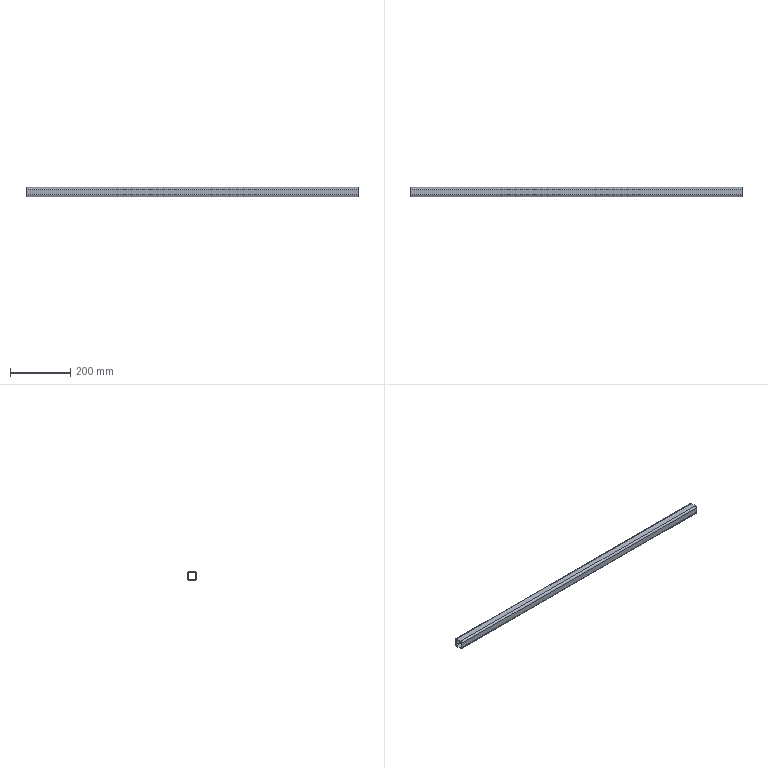Component | SolidWorks | 30X30X3-1100-3 | 1 solid | 18 faces | box 1100 x 30 x 30 mm | volume 330905 mm3 | plane 10 | cylinder 8 | commonest cylinder face diameters 12 x4 6 x4
build123d program:
from build123d import *

# Parameters (mm, degrees)
GB_6728_1986_SQUARE_HOLLOW_SECTION_030_X_DEPTH = 1100


with BuildPart() as part:
    # Sketch1 → Gb_6728-1986 Square Hollow Section 030 X (new body)
    with BuildSketch(Plane(origin=(0, 0, 0), x_dir=(-1, 0, 0), z_dir=(0, 1, 0))):
        with BuildLine():
            Line((-9, -15), (9, -15))
            ThreePointArc((9, -15), (13.243, -13.243), (15, -9))
            Line((15, -9), (15, 9))
            ThreePointArc((15, 9), (13.243, 13.243), (9, 15))
            Line((9, 15), (-9, 15))
            ThreePointArc((-9, 15), (-13.243, 13.243), (-15, 9))
            Line((-15, 9), (-15, -9))
            ThreePointArc((-15, -9), (-13.243, -13.243), (-9, -15))
        make_face()
        with BuildLine():
            Line((-9, -12), (9, -12))
            ThreePointArc((9, -12), (11.121, -11.121), (12, -9))
            Line((12, -9), (12, 9))
            ThreePointArc((12, 9), (11.121, 11.121), (9, 12))
            Line((9, 12), (-9, 12))
            ThreePointArc((-9, 12), (-11.121, 11.121), (-12, 9))
            Line((-12, 9), (-12, -9))
            ThreePointArc((-12, -9), (-11.121, -11.121), (-9, -12))
        make_face(mode=Mode.SUBTRACT)
    extrude(amount=GB_6728_1986_SQUARE_HOLLOW_SECTION_030_X_DEPTH)


solid = part.part

# Placed as in the assembly
solid = solid.moved(Location((3169.926, -31179.846, 5264), (0, 0, 90)))
STEP:
#1=COLOUR_RGB('',0.7922,0.8196,0.9333);
#2=FILL_AREA_STYLE_COLOUR('',#1);
#3=FILL_AREA_STYLE('',(#2));
#4=SURFACE_STYLE_FILL_AREA(#3);
#5=SURFACE_SIDE_STYLE('',(#4));
#6=SURFACE_STYLE_USAGE(.BOTH.,#5);
#7=PRESENTATION_STYLE_ASSIGNMENT((#6));
#8=CARTESIAN_POINT('',(81.493,-1227.199,206.654));
#9=VERTEX_POINT('',#8);
#10=CARTESIAN_POINT('',(81.493,-1226.962,206.89));
#11=VERTEX_POINT('',#10);
#12=CARTESIAN_POINT('',(81.493,-1227.199,206.89));
#13=DIRECTION('',(1.,-0.,-0.));
#14=DIRECTION('',(0.,1.,0.));
#15=AXIS2_PLACEMENT_3D('',#12,#13,#14);
#16=CIRCLE('',#15,0.2362);
#17=EDGE_CURVE('',#9,#11,#16,.T.);
#18=ORIENTED_EDGE('',*,*,#17,.T.);
#19=CARTESIAN_POINT('',(124.8,-1226.962,206.89));
#20=VERTEX_POINT('',#19);
#21=CARTESIAN_POINT('',(124.8,-1226.962,206.89));
#22=DIRECTION('',(-1.,0.,0.));
#23=VECTOR('',#22,39.37);
#24=LINE('',#21,#23);
#25=EDGE_CURVE('',#20,#11,#24,.T.);
#26=ORIENTED_EDGE('',*,*,#25,.F.);
#27=CARTESIAN_POINT('',(124.8,-1227.199,206.654));
#28=VERTEX_POINT('',#27);
#29=CARTESIAN_POINT('',(124.8,-1227.199,206.89));
#30=DIRECTION('',(1.,-0.,-0.));
#31=DIRECTION('',(0.,1.,0.));
#32=AXIS2_PLACEMENT_3D('',#29,#30,#31);
#33=CIRCLE('',#32,0.2362);
#34=EDGE_CURVE('',#28,#20,#33,.T.);
#35=ORIENTED_EDGE('',*,*,#34,.F.);
#36=CARTESIAN_POINT('',(124.8,-1227.199,206.654));
#37=DIRECTION('',(-1.,0.,0.));
#38=VECTOR('',#37,39.37);
#39=LINE('',#36,#38);
#40=EDGE_CURVE('',#28,#9,#39,.T.);
#41=ORIENTED_EDGE('',*,*,#40,.T.);
#42=EDGE_LOOP('',(#18,#26,#35,#41));
#43=FACE_OUTER_BOUND('',#42,.T.);
#44=CARTESIAN_POINT('',(124.8,-1227.199,206.89));
#45=DIRECTION('',(-1.,0.,0.));
#46=DIRECTION('',(0.,-1.,0.));
#47=AXIS2_PLACEMENT_3D('',#44,#45,#46);
#48=CYLINDRICAL_SURFACE('',#47,0.2362);
#49=ADVANCED_FACE('',(#43),#48,.T.);
#50=CARTESIAN_POINT('',(81.493,-1226.962,207.598));
#51=VERTEX_POINT('',#50);
#52=CARTESIAN_POINT('',(81.493,-1226.962,206.89));
#53=DIRECTION('',(0.,-0.,1.));
#54=VECTOR('',#53,39.37);
#55=LINE('',#52,#54);
#56=EDGE_CURVE('',#11,#51,#55,.T.);
#57=ORIENTED_EDGE('',*,*,#56,.T.);
#58=CARTESIAN_POINT('',(124.8,-1226.962,207.598));
#59=VERTEX_POINT('',#58);
#60=CARTESIAN_POINT('',(124.8,-1226.962,207.598));
#61=DIRECTION('',(-1.,0.,0.));
#62=VECTOR('',#61,39.37);
#63=LINE('',#60,#62);
#64=EDGE_CURVE('',#59,#51,#63,.T.);
#65=ORIENTED_EDGE('',*,*,#64,.F.);
#66=CARTESIAN_POINT('',(124.8,-1226.962,206.89));
#67=DIRECTION('',(0.,-0.,1.));
#68=VECTOR('',#67,39.37);
#69=LINE('',#66,#68);
#70=EDGE_CURVE('',#20,#59,#69,.T.);
#71=ORIENTED_EDGE('',*,*,#70,.F.);
#72=ORIENTED_EDGE('',*,*,#25,.T.);
#73=EDGE_LOOP('',(#57,#65,#71,#72));
#74=FACE_OUTER_BOUND('',#73,.T.);
#75=CARTESIAN_POINT('',(124.8,-1226.962,206.89));
#76=DIRECTION('',(-0.,-1.,-0.));
#77=DIRECTION('',(-0.,0.,-1.));
#78=AXIS2_PLACEMENT_3D('',#75,#76,#77);
#79=PLANE('',#78);
#80=ADVANCED_FACE('',(#74),#79,.F.);
#81=CARTESIAN_POINT('',(81.493,-1227.199,207.835));
#82=VERTEX_POINT('',#81);
#83=CARTESIAN_POINT('',(81.493,-1227.199,207.598));
#84=DIRECTION('',(1.,-0.,-0.));
#85=DIRECTION('',(0.,1.,0.));
#86=AXIS2_PLACEMENT_3D('',#83,#84,#85);
#87=CIRCLE('',#86,0.2362);
#88=EDGE_CURVE('',#51,#82,#87,.T.);
#89=ORIENTED_EDGE('',*,*,#88,.T.);
#90=CARTESIAN_POINT('',(124.8,-1227.199,207.835));
#91=VERTEX_POINT('',#90);
#92=CARTESIAN_POINT('',(124.8,-1227.199,207.835));
#93=DIRECTION('',(-1.,0.,0.));
#94=VECTOR('',#93,39.37);
#95=LINE('',#92,#94);
#96=EDGE_CURVE('',#91,#82,#95,.T.);
#97=ORIENTED_EDGE('',*,*,#96,.F.);
#98=CARTESIAN_POINT('',(124.8,-1227.199,207.598));
#99=DIRECTION('',(1.,-0.,-0.));
#100=DIRECTION('',(0.,1.,0.));
#101=AXIS2_PLACEMENT_3D('',#98,#99,#100);
#102=CIRCLE('',#101,0.2362);
#103=EDGE_CURVE('',#59,#91,#102,.T.);
#104=ORIENTED_EDGE('',*,*,#103,.F.);
#105=ORIENTED_EDGE('',*,*,#64,.T.);
#106=EDGE_LOOP('',(#89,#97,#104,#105));
#107=FACE_OUTER_BOUND('',#106,.T.);
#108=CARTESIAN_POINT('',(124.8,-1227.199,207.598));
#109=DIRECTION('',(-1.,0.,0.));
#110=DIRECTION('',(0.,-1.,0.));
#111=AXIS2_PLACEMENT_3D('',#108,#109,#110);
#112=CYLINDRICAL_SURFACE('',#111,0.2362);
#113=ADVANCED_FACE('',(#107),#112,.T.);
#114=CARTESIAN_POINT('',(81.493,-1227.907,207.835));
#115=VERTEX_POINT('',#114);
#116=CARTESIAN_POINT('',(81.493,-1227.907,207.835));
#117=DIRECTION('',(-0.,-1.,-0.));
#118=VECTOR('',#117,39.37);
#119=LINE('',#116,#118);
#120=EDGE_CURVE('',#82,#115,#119,.T.);
#121=ORIENTED_EDGE('',*,*,#120,.T.);
#122=CARTESIAN_POINT('',(124.8,-1227.907,207.835));
#123=VERTEX_POINT('',#122);
#124=CARTESIAN_POINT('',(124.8,-1227.907,207.835));
#125=DIRECTION('',(-1.,0.,0.));
#126=VECTOR('',#125,39.37);
#127=LINE('',#124,#126);
#128=EDGE_CURVE('',#123,#115,#127,.T.);
#129=ORIENTED_EDGE('',*,*,#128,.F.);
#130=CARTESIAN_POINT('',(124.8,-1227.907,207.835));
#131=DIRECTION('',(-0.,-1.,-0.));
#132=VECTOR('',#131,39.37);
#133=LINE('',#130,#132);
#134=EDGE_CURVE('',#91,#123,#133,.T.);
#135=ORIENTED_EDGE('',*,*,#134,.F.);
#136=ORIENTED_EDGE('',*,*,#96,.T.);
#137=EDGE_LOOP('',(#121,#129,#135,#136));
#138=FACE_OUTER_BOUND('',#137,.T.);
#139=CARTESIAN_POINT('',(124.8,-1227.907,207.835));
#140=DIRECTION('',(-0.,0.,-1.));
#141=DIRECTION('',(0.,1.,0.));
#142=AXIS2_PLACEMENT_3D('',#139,#140,#141);
#143=PLANE('',#142);
#144=ADVANCED_FACE('',(#138),#143,.F.);
#145=CARTESIAN_POINT('',(81.493,-1228.144,207.598));
#146=VERTEX_POINT('',#145);
#147=CARTESIAN_POINT('',(81.493,-1227.907,207.598));
#148=DIRECTION('',(1.,-0.,-0.));
#149=DIRECTION('',(0.,1.,0.));
#150=AXIS2_PLACEMENT_3D('',#147,#148,#149);
#151=CIRCLE('',#150,0.2362);
#152=EDGE_CURVE('',#115,#146,#151,.T.);
#153=ORIENTED_EDGE('',*,*,#152,.T.);
#154=CARTESIAN_POINT('',(124.8,-1228.144,207.598));
#155=VERTEX_POINT('',#154);
#156=CARTESIAN_POINT('',(124.8,-1228.144,207.598));
#157=DIRECTION('',(-1.,0.,0.));
#158=VECTOR('',#157,39.37);
#159=LINE('',#156,#158);
#160=EDGE_CURVE('',#155,#146,#159,.T.);
#161=ORIENTED_EDGE('',*,*,#160,.F.);
#162=CARTESIAN_POINT('',(124.8,-1227.907,207.598));
#163=DIRECTION('',(1.,-0.,-0.));
#164=DIRECTION('',(0.,1.,0.));
#165=AXIS2_PLACEMENT_3D('',#162,#163,#164);
#166=CIRCLE('',#165,0.2362);
#167=EDGE_CURVE('',#123,#155,#166,.T.);
#168=ORIENTED_EDGE('',*,*,#167,.F.);
#169=ORIENTED_EDGE('',*,*,#128,.T.);
#170=EDGE_LOOP('',(#153,#161,#168,#169));
#171=FACE_OUTER_BOUND('',#170,.T.);
#172=CARTESIAN_POINT('',(124.8,-1227.907,207.598));
#173=DIRECTION('',(-1.,0.,0.));
#174=DIRECTION('',(0.,-1.,0.));
#175=AXIS2_PLACEMENT_3D('',#172,#173,#174);
#176=CYLINDRICAL_SURFACE('',#175,0.2362);
#177=ADVANCED_FACE('',(#171),#176,.T.);
#178=CARTESIAN_POINT('',(81.493,-1228.144,206.89));
#179=VERTEX_POINT('',#178);
#180=CARTESIAN_POINT('',(81.493,-1228.144,207.598));
#181=DIRECTION('',(-0.,0.,-1.));
#182=VECTOR('',#181,39.37);
#183=LINE('',#180,#182);
#184=EDGE_CURVE('',#146,#179,#183,.T.);
#185=ORIENTED_EDGE('',*,*,#184,.T.);
#186=CARTESIAN_POINT('',(124.8,-1228.144,206.89));
#187=VERTEX_POINT('',#186);
#188=CARTESIAN_POINT('',(124.8,-1228.144,206.89));
#189=DIRECTION('',(-1.,0.,0.));
#190=VECTOR('',#189,39.37);
#191=LINE('',#188,#190);
#192=EDGE_CURVE('',#187,#179,#191,.T.);
#193=ORIENTED_EDGE('',*,*,#192,.F.);
#194=CARTESIAN_POINT('',(124.8,-1228.144,207.598));
#195=DIRECTION('',(-0.,0.,-1.));
#196=VECTOR('',#195,39.37);
#197=LINE('',#194,#196);
#198=EDGE_CURVE('',#155,#187,#197,.T.);
#199=ORIENTED_EDGE('',*,*,#198,.F.);
#200=ORIENTED_EDGE('',*,*,#160,.T.);
#201=EDGE_LOOP('',(#185,#193,#199,#200));
#202=FACE_OUTER_BOUND('',#201,.T.);
#203=CARTESIAN_POINT('',(124.8,-1228.144,207.598));
#204=DIRECTION('',(0.,1.,0.));
#205=DIRECTION('',(0.,-0.,1.));
#206=AXIS2_PLACEMENT_3D('',#203,#204,#205);
#207=PLANE('',#206);
#208=ADVANCED_FACE('',(#202),#207,.F.);
#209=CARTESIAN_POINT('',(81.493,-1227.907,206.654));
#210=VERTEX_POINT('',#209);
#211=CARTESIAN_POINT('',(81.493,-1227.907,206.89));
#212=DIRECTION('',(1.,-0.,-0.));
#213=DIRECTION('',(0.,1.,0.));
#214=AXIS2_PLACEMENT_3D('',#211,#212,#213);
#215=CIRCLE('',#214,0.2362);
#216=EDGE_CURVE('',#179,#210,#215,.T.);
#217=ORIENTED_EDGE('',*,*,#216,.T.);
#218=CARTESIAN_POINT('',(124.8,-1227.907,206.654));
#219=VERTEX_POINT('',#218);
#220=CARTESIAN_POINT('',(124.8,-1227.907,206.654));
#221=DIRECTION('',(-1.,0.,0.));
#222=VECTOR('',#221,39.37);
#223=LINE('',#220,#222);
#224=EDGE_CURVE('',#219,#210,#223,.T.);
#225=ORIENTED_EDGE('',*,*,#224,.F.);
#226=CARTESIAN_POINT('',(124.8,-1227.907,206.89));
#227=DIRECTION('',(1.,-0.,-0.));
#228=DIRECTION('',(0.,1.,0.));
#229=AXIS2_PLACEMENT_3D('',#226,#227,#228);
#230=CIRCLE('',#229,0.2362);
#231=EDGE_CURVE('',#187,#219,#230,.T.);
#232=ORIENTED_EDGE('',*,*,#231,.F.);
#233=ORIENTED_EDGE('',*,*,#192,.T.);
#234=EDGE_LOOP('',(#217,#225,#232,#233));
#235=FACE_OUTER_BOUND('',#234,.T.);
#236=CARTESIAN_POINT('',(124.8,-1227.907,206.89));
#237=DIRECTION('',(-1.,0.,0.));
#238=DIRECTION('',(0.,-1.,0.));
#239=AXIS2_PLACEMENT_3D('',#236,#237,#238);
#240=CYLINDRICAL_SURFACE('',#239,0.2362);
#241=ADVANCED_FACE('',(#235),#240,.T.);
#242=CARTESIAN_POINT('',(81.493,-1227.081,207.598));
#243=VERTEX_POINT('',#242);
#244=CARTESIAN_POINT('',(81.493,-1227.199,207.717));
#245=VERTEX_POINT('',#244);
#246=CARTESIAN_POINT('',(81.493,-1227.199,207.598));
#247=DIRECTION('',(1.,-0.,-0.));
#248=DIRECTION('',(0.,1.,0.));
#249=AXIS2_PLACEMENT_3D('',#246,#247,#248);
#250=CIRCLE('',#249,0.1181);
#251=EDGE_CURVE('',#243,#245,#250,.T.);
#252=ORIENTED_EDGE('',*,*,#251,.F.);
#253=CARTESIAN_POINT('',(124.8,-1227.081,207.598));
#254=VERTEX_POINT('',#253);
#255=CARTESIAN_POINT('',(124.8,-1227.081,207.598));
#256=DIRECTION('',(-1.,0.,0.));
#257=VECTOR('',#256,39.37);
#258=LINE('',#255,#257);
#259=EDGE_CURVE('',#254,#243,#258,.T.);
#260=ORIENTED_EDGE('',*,*,#259,.F.);
#261=CARTESIAN_POINT('',(124.8,-1227.199,207.717));
#262=VERTEX_POINT('',#261);
#263=CARTESIAN_POINT('',(124.8,-1227.199,207.598));
#264=DIRECTION('',(1.,-0.,-0.));
#265=DIRECTION('',(0.,1.,0.));
#266=AXIS2_PLACEMENT_3D('',#263,#264,#265);
#267=CIRCLE('',#266,0.1181);
#268=EDGE_CURVE('',#254,#262,#267,.T.);
#269=ORIENTED_EDGE('',*,*,#268,.T.);
#270=CARTESIAN_POINT('',(124.8,-1227.199,207.717));
#271=DIRECTION('',(-1.,0.,0.));
#272=VECTOR('',#271,39.37);
#273=LINE('',#270,#272);
#274=EDGE_CURVE('',#262,#245,#273,.T.);
#275=ORIENTED_EDGE('',*,*,#274,.T.);
#276=EDGE_LOOP('',(#252,#260,#269,#275));
#277=FACE_OUTER_BOUND('',#276,.T.);
#278=CARTESIAN_POINT('',(124.8,-1227.199,207.598));
#279=DIRECTION('',(-1.,0.,0.));
#280=DIRECTION('',(0.,-1.,0.));
#281=AXIS2_PLACEMENT_3D('',#278,#279,#280);
#282=CYLINDRICAL_SURFACE('',#281,0.1181);
#283=ADVANCED_FACE('',(#277),#282,.F.);
#284=CARTESIAN_POINT('',(81.493,-1227.081,206.89));
#285=VERTEX_POINT('',#284);
#286=CARTESIAN_POINT('',(81.493,-1227.081,206.89));
#287=DIRECTION('',(0.,-0.,1.));
#288=VECTOR('',#287,39.37);
#289=LINE('',#286,#288);
#290=EDGE_CURVE('',#285,#243,#289,.T.);
#291=ORIENTED_EDGE('',*,*,#290,.F.);
#292=CARTESIAN_POINT('',(124.8,-1227.081,206.89));
#293=VERTEX_POINT('',#292);
#294=CARTESIAN_POINT('',(124.8,-1227.081,206.89));
#295=DIRECTION('',(-1.,0.,0.));
#296=VECTOR('',#295,39.37);
#297=LINE('',#294,#296);
#298=EDGE_CURVE('',#293,#285,#297,.T.);
#299=ORIENTED_EDGE('',*,*,#298,.F.);
#300=CARTESIAN_POINT('',(124.8,-1227.081,206.89));
#301=DIRECTION('',(0.,-0.,1.));
#302=VECTOR('',#301,39.37);
#303=LINE('',#300,#302);
#304=EDGE_CURVE('',#293,#254,#303,.T.);
#305=ORIENTED_EDGE('',*,*,#304,.T.);
#306=ORIENTED_EDGE('',*,*,#259,.T.);
#307=EDGE_LOOP('',(#291,#299,#305,#306));
#308=FACE_OUTER_BOUND('',#307,.T.);
#309=CARTESIAN_POINT('',(124.8,-1227.081,206.89));
#310=DIRECTION('',(-0.,-1.,-0.));
#311=DIRECTION('',(-0.,0.,-1.));
#312=AXIS2_PLACEMENT_3D('',#309,#310,#311);
#313=PLANE('',#312);
#314=ADVANCED_FACE('',(#308),#313,.T.);
#315=CARTESIAN_POINT('',(81.493,-1227.199,206.772));
#316=VERTEX_POINT('',#315);
#317=CARTESIAN_POINT('',(81.493,-1227.199,206.89));
#318=DIRECTION('',(1.,-0.,-0.));
#319=DIRECTION('',(0.,1.,0.));
#320=AXIS2_PLACEMENT_3D('',#317,#318,#319);
#321=CIRCLE('',#320,0.1181);
#322=EDGE_CURVE('',#316,#285,#321,.T.);
#323=ORIENTED_EDGE('',*,*,#322,.F.);
#324=CARTESIAN_POINT('',(124.8,-1227.199,206.772));
#325=VERTEX_POINT('',#324);
#326=CARTESIAN_POINT('',(124.8,-1227.199,206.772));
#327=DIRECTION('',(-1.,0.,0.));
#328=VECTOR('',#327,39.37);
#329=LINE('',#326,#328);
#330=EDGE_CURVE('',#325,#316,#329,.T.);
#331=ORIENTED_EDGE('',*,*,#330,.F.);
#332=CARTESIAN_POINT('',(124.8,-1227.199,206.89));
#333=DIRECTION('',(1.,-0.,-0.));
#334=DIRECTION('',(0.,1.,0.));
#335=AXIS2_PLACEMENT_3D('',#332,#333,#334);
#336=CIRCLE('',#335,0.1181);
#337=EDGE_CURVE('',#325,#293,#336,.T.);
#338=ORIENTED_EDGE('',*,*,#337,.T.);
#339=ORIENTED_EDGE('',*,*,#298,.T.);
#340=EDGE_LOOP('',(#323,#331,#338,#339));
#341=FACE_OUTER_BOUND('',#340,.T.);
#342=CARTESIAN_POINT('',(124.8,-1227.199,206.89));
#343=DIRECTION('',(-1.,0.,0.));
#344=DIRECTION('',(0.,-1.,0.));
#345=AXIS2_PLACEMENT_3D('',#342,#343,#344);
#346=CYLINDRICAL_SURFACE('',#345,0.1181);
#347=ADVANCED_FACE('',(#341),#346,.F.);
#348=CARTESIAN_POINT('',(81.493,-1227.907,206.772));
#349=VERTEX_POINT('',#348);
#350=CARTESIAN_POINT('',(81.493,-1227.199,206.772));
#351=DIRECTION('',(0.,1.,0.));
#352=VECTOR('',#351,39.37);
#353=LINE('',#350,#352);
#354=EDGE_CURVE('',#349,#316,#353,.T.);
#355=ORIENTED_EDGE('',*,*,#354,.F.);
#356=CARTESIAN_POINT('',(124.8,-1227.907,206.772));
#357=VERTEX_POINT('',#356);
#358=CARTESIAN_POINT('',(124.8,-1227.907,206.772));
#359=DIRECTION('',(-1.,0.,0.));
#360=VECTOR('',#359,39.37);
#361=LINE('',#358,#360);
#362=EDGE_CURVE('',#357,#349,#361,.T.);
#363=ORIENTED_EDGE('',*,*,#362,.F.);
#364=CARTESIAN_POINT('',(124.8,-1227.199,206.772));
#365=DIRECTION('',(0.,1.,0.));
#366=VECTOR('',#365,39.37);
#367=LINE('',#364,#366);
#368=EDGE_CURVE('',#357,#325,#367,.T.);
#369=ORIENTED_EDGE('',*,*,#368,.T.);
#370=ORIENTED_EDGE('',*,*,#330,.T.);
#371=EDGE_LOOP('',(#355,#363,#369,#370));
#372=FACE_OUTER_BOUND('',#371,.T.);
#373=CARTESIAN_POINT('',(124.8,-1227.199,206.772));
#374=DIRECTION('',(0.,-0.,1.));
#375=DIRECTION('',(-0.,-1.,-0.));
#376=AXIS2_PLACEMENT_3D('',#373,#374,#375);
#377=PLANE('',#376);
#378=ADVANCED_FACE('',(#372),#377,.T.);
#379=CARTESIAN_POINT('',(81.493,-1228.025,206.89));
#380=VERTEX_POINT('',#379);
#381=CARTESIAN_POINT('',(81.493,-1227.907,206.89));
#382=DIRECTION('',(1.,-0.,-0.));
#383=DIRECTION('',(0.,1.,0.));
#384=AXIS2_PLACEMENT_3D('',#381,#382,#383);
#385=CIRCLE('',#384,0.1181);
#386=EDGE_CURVE('',#380,#349,#385,.T.);
#387=ORIENTED_EDGE('',*,*,#386,.F.);
#388=CARTESIAN_POINT('',(124.8,-1228.025,206.89));
#389=VERTEX_POINT('',#388);
#390=CARTESIAN_POINT('',(124.8,-1228.025,206.89));
#391=DIRECTION('',(-1.,0.,0.));
#392=VECTOR('',#391,39.37);
#393=LINE('',#390,#392);
#394=EDGE_CURVE('',#389,#380,#393,.T.);
#395=ORIENTED_EDGE('',*,*,#394,.F.);
#396=CARTESIAN_POINT('',(124.8,-1227.907,206.89));
#397=DIRECTION('',(1.,-0.,-0.));
#398=DIRECTION('',(0.,1.,0.));
#399=AXIS2_PLACEMENT_3D('',#396,#397,#398);
#400=CIRCLE('',#399,0.1181);
#401=EDGE_CURVE('',#389,#357,#400,.T.);
#402=ORIENTED_EDGE('',*,*,#401,.T.);
#403=ORIENTED_EDGE('',*,*,#362,.T.);
#404=EDGE_LOOP('',(#387,#395,#402,#403));
#405=FACE_OUTER_BOUND('',#404,.T.);
#406=CARTESIAN_POINT('',(124.8,-1227.907,206.89));
#407=DIRECTION('',(-1.,0.,0.));
#408=DIRECTION('',(0.,-1.,0.));
#409=AXIS2_PLACEMENT_3D('',#406,#407,#408);
#410=CYLINDRICAL_SURFACE('',#409,0.1181);
#411=ADVANCED_FACE('',(#405),#410,.F.);
#412=CARTESIAN_POINT('',(81.493,-1228.025,207.598));
#413=VERTEX_POINT('',#412);
#414=CARTESIAN_POINT('',(81.493,-1228.025,207.598));
#415=DIRECTION('',(-0.,0.,-1.));
#416=VECTOR('',#415,39.37);
#417=LINE('',#414,#416);
#418=EDGE_CURVE('',#413,#380,#417,.T.);
#419=ORIENTED_EDGE('',*,*,#418,.F.);
#420=CARTESIAN_POINT('',(124.8,-1228.025,207.598));
#421=VERTEX_POINT('',#420);
#422=CARTESIAN_POINT('',(124.8,-1228.025,207.598));
#423=DIRECTION('',(-1.,0.,0.));
#424=VECTOR('',#423,39.37);
#425=LINE('',#422,#424);
#426=EDGE_CURVE('',#421,#413,#425,.T.);
#427=ORIENTED_EDGE('',*,*,#426,.F.);
#428=CARTESIAN_POINT('',(124.8,-1228.025,207.598));
#429=DIRECTION('',(-0.,0.,-1.));
#430=VECTOR('',#429,39.37);
#431=LINE('',#428,#430);
#432=EDGE_CURVE('',#421,#389,#431,.T.);
#433=ORIENTED_EDGE('',*,*,#432,.T.);
#434=ORIENTED_EDGE('',*,*,#394,.T.);
#435=EDGE_LOOP('',(#419,#427,#433,#434));
#436=FACE_OUTER_BOUND('',#435,.T.);
#437=CARTESIAN_POINT('',(124.8,-1228.025,207.598));
#438=DIRECTION('',(0.,1.,0.));
#439=DIRECTION('',(0.,-0.,1.));
#440=AXIS2_PLACEMENT_3D('',#437,#438,#439);
#441=PLANE('',#440);
#442=ADVANCED_FACE('',(#436),#441,.T.);
#443=CARTESIAN_POINT('',(81.493,-1227.907,207.717));
#444=VERTEX_POINT('',#443);
#445=CARTESIAN_POINT('',(81.493,-1227.907,207.598));
#446=DIRECTION('',(1.,-0.,-0.));
#447=DIRECTION('',(0.,1.,0.));
#448=AXIS2_PLACEMENT_3D('',#445,#446,#447);
#449=CIRCLE('',#448,0.1181);
#450=EDGE_CURVE('',#444,#413,#449,.T.);
#451=ORIENTED_EDGE('',*,*,#450,.F.);
#452=CARTESIAN_POINT('',(124.8,-1227.907,207.717));
#453=VERTEX_POINT('',#452);
#454=CARTESIAN_POINT('',(124.8,-1227.907,207.717));
#455=DIRECTION('',(-1.,0.,0.));
#456=VECTOR('',#455,39.37);
#457=LINE('',#454,#456);
#458=EDGE_CURVE('',#453,#444,#457,.T.);
#459=ORIENTED_EDGE('',*,*,#458,.F.);
#460=CARTESIAN_POINT('',(124.8,-1227.907,207.598));
#461=DIRECTION('',(1.,-0.,-0.));
#462=DIRECTION('',(0.,1.,0.));
#463=AXIS2_PLACEMENT_3D('',#460,#461,#462);
#464=CIRCLE('',#463,0.1181);
#465=EDGE_CURVE('',#453,#421,#464,.T.);
#466=ORIENTED_EDGE('',*,*,#465,.T.);
#467=ORIENTED_EDGE('',*,*,#426,.T.);
#468=EDGE_LOOP('',(#451,#459,#466,#467));
#469=FACE_OUTER_BOUND('',#468,.T.);
#470=CARTESIAN_POINT('',(124.8,-1227.907,207.598));
#471=DIRECTION('',(-1.,0.,0.));
#472=DIRECTION('',(0.,-1.,0.));
#473=AXIS2_PLACEMENT_3D('',#470,#471,#472);
#474=CYLINDRICAL_SURFACE('',#473,0.1181);
#475=ADVANCED_FACE('',(#469),#474,.F.);
#476=CARTESIAN_POINT('',(81.493,-1227.907,207.717));
#477=DIRECTION('',(-0.,-1.,-0.));
#478=VECTOR('',#477,39.37);
#479=LINE('',#476,#478);
#480=EDGE_CURVE('',#245,#444,#479,.T.);
#481=ORIENTED_EDGE('',*,*,#480,.F.);
#482=ORIENTED_EDGE('',*,*,#274,.F.);
#483=CARTESIAN_POINT('',(124.8,-1227.907,207.717));
#484=DIRECTION('',(-0.,-1.,-0.));
#485=VECTOR('',#484,39.37);
#486=LINE('',#483,#485);
#487=EDGE_CURVE('',#262,#453,#486,.T.);
#488=ORIENTED_EDGE('',*,*,#487,.T.);
#489=ORIENTED_EDGE('',*,*,#458,.T.);
#490=EDGE_LOOP('',(#481,#482,#488,#489));
#491=FACE_OUTER_BOUND('',#490,.T.);
#492=CARTESIAN_POINT('',(124.8,-1227.907,207.717));
#493=DIRECTION('',(-0.,0.,-1.));
#494=DIRECTION('',(0.,1.,0.));
#495=AXIS2_PLACEMENT_3D('',#492,#493,#494);
#496=PLANE('',#495);
#497=ADVANCED_FACE('',(#491),#496,.T.);
#498=CARTESIAN_POINT('',(81.493,-1227.199,206.654));
#499=DIRECTION('',(0.,1.,0.));
#500=VECTOR('',#499,39.37);
#501=LINE('',#498,#500);
#502=EDGE_CURVE('',#210,#9,#501,.T.);
#503=ORIENTED_EDGE('',*,*,#502,.T.);
#504=ORIENTED_EDGE('',*,*,#40,.F.);
#505=CARTESIAN_POINT('',(124.8,-1227.199,206.654));
#506=DIRECTION('',(0.,1.,0.));
#507=VECTOR('',#506,39.37);
#508=LINE('',#505,#507);
#509=EDGE_CURVE('',#219,#28,#508,.T.);
#510=ORIENTED_EDGE('',*,*,#509,.F.);
#511=ORIENTED_EDGE('',*,*,#224,.T.);
#512=EDGE_LOOP('',(#503,#504,#510,#511));
#513=FACE_OUTER_BOUND('',#512,.T.);
#514=CARTESIAN_POINT('',(124.8,-1227.199,206.654));
#515=DIRECTION('',(0.,-0.,1.));
#516=DIRECTION('',(-0.,-1.,-0.));
#517=AXIS2_PLACEMENT_3D('',#514,#515,#516);
#518=PLANE('',#517);
#519=ADVANCED_FACE('',(#513),#518,.F.);
#520=ORIENTED_EDGE('',*,*,#268,.F.);
#521=ORIENTED_EDGE('',*,*,#304,.F.);
#522=ORIENTED_EDGE('',*,*,#337,.F.);
#523=ORIENTED_EDGE('',*,*,#368,.F.);
#524=ORIENTED_EDGE('',*,*,#401,.F.);
#525=ORIENTED_EDGE('',*,*,#432,.F.);
#526=ORIENTED_EDGE('',*,*,#465,.F.);
#527=ORIENTED_EDGE('',*,*,#487,.F.);
#528=EDGE_LOOP('',(#520,#521,#522,#523,#524,#525,#526,#527));
#529=FACE_BOUND('',#528,.T.);
#530=ORIENTED_EDGE('',*,*,#34,.T.);
#531=ORIENTED_EDGE('',*,*,#70,.T.);
#532=ORIENTED_EDGE('',*,*,#103,.T.);
#533=ORIENTED_EDGE('',*,*,#134,.T.);
#534=ORIENTED_EDGE('',*,*,#167,.T.);
#535=ORIENTED_EDGE('',*,*,#198,.T.);
#536=ORIENTED_EDGE('',*,*,#231,.T.);
#537=ORIENTED_EDGE('',*,*,#509,.T.);
#538=EDGE_LOOP('',(#530,#531,#532,#533,#534,#535,#536,#537));
#539=FACE_OUTER_BOUND('',#538,.T.);
#540=CARTESIAN_POINT('',(124.8,-1227.199,206.89));
#541=DIRECTION('',(1.,-0.,-0.));
#542=DIRECTION('',(0.,1.,0.));
#543=AXIS2_PLACEMENT_3D('',#540,#541,#542);
#544=PLANE('',#543);
#545=ADVANCED_FACE('',(#529,#539),#544,.T.);
#546=ORIENTED_EDGE('',*,*,#251,.T.);
#547=ORIENTED_EDGE('',*,*,#480,.T.);
#548=ORIENTED_EDGE('',*,*,#450,.T.);
#549=ORIENTED_EDGE('',*,*,#418,.T.);
#550=ORIENTED_EDGE('',*,*,#386,.T.);
#551=ORIENTED_EDGE('',*,*,#354,.T.);
#552=ORIENTED_EDGE('',*,*,#322,.T.);
#553=ORIENTED_EDGE('',*,*,#290,.T.);
#554=EDGE_LOOP('',(#546,#547,#548,#549,#550,#551,#552,#553));
#555=FACE_BOUND('',#554,.T.);
#556=ORIENTED_EDGE('',*,*,#17,.F.);
#557=ORIENTED_EDGE('',*,*,#502,.F.);
#558=ORIENTED_EDGE('',*,*,#216,.F.);
#559=ORIENTED_EDGE('',*,*,#184,.F.);
#560=ORIENTED_EDGE('',*,*,#152,.F.);
#561=ORIENTED_EDGE('',*,*,#120,.F.);
#562=ORIENTED_EDGE('',*,*,#88,.F.);
#563=ORIENTED_EDGE('',*,*,#56,.F.);
#564=EDGE_LOOP('',(#556,#557,#558,#559,#560,#561,#562,#563));
#565=FACE_OUTER_BOUND('',#564,.T.);
#566=CARTESIAN_POINT('',(81.493,-1227.199,206.89));
#567=DIRECTION('',(1.,-0.,-0.));
#568=DIRECTION('',(0.,1.,0.));
#569=AXIS2_PLACEMENT_3D('',#566,#567,#568);
#570=PLANE('',#569);
#571=ADVANCED_FACE('',(#555,#565),#570,.F.);
#572=CLOSED_SHELL('',(#49,#80,#113,#144,#177,#208,#241,#283,#314,#347,#378,#411,#442,#475,#497,#519,#545,#571));
#573=MANIFOLD_SOLID_BREP('',#572);
#574=STYLED_ITEM('',(#7),#573);
#575=(LENGTH_UNIT()NAMED_UNIT(*)SI_UNIT($,.METRE.));
#576=LENGTH_MEASURE_WITH_UNIT(LENGTH_MEASURE(0.0254),#575);
#577=DIMENSIONAL_EXPONENTS(1.,0.,0.,0.,0.,0.,0.);
#578=(CONVERSION_BASED_UNIT('',#576)LENGTH_UNIT()NAMED_UNIT(#577));
#579=UNCERTAINTY_MEASURE_WITH_UNIT(LENGTH_MEASURE(0.00001),#578,'','');
#580=(NAMED_UNIT(*)PLANE_ANGLE_UNIT()SI_UNIT($,.RADIAN.));
#581=(NAMED_UNIT(*)SI_UNIT($,.STERADIAN.)SOLID_ANGLE_UNIT());
#582=(GEOMETRIC_REPRESENTATION_CONTEXT(3)GLOBAL_UNCERTAINTY_ASSIGNED_CONTEXT((#579))GLOBAL_UNIT_ASSIGNED_CONTEXT((#578,#580,#581))REPRESENTATION_CONTEXT('',''));
#583=MECHANICAL_DESIGN_GEOMETRIC_PRESENTATION_REPRESENTATION('',(#574),#582);
#584=CARTESIAN_POINT('',(0.,0.,0.));
#585=DIRECTION('',(0.,0.,1.));
#586=DIRECTION('',(1.,0.,0.));
#587=AXIS2_PLACEMENT_3D('',#584,#585,#586);
#588=(LENGTH_UNIT()NAMED_UNIT(*)SI_UNIT($,.METRE.));
#589=LENGTH_MEASURE_WITH_UNIT(LENGTH_MEASURE(0.0254),#588);
#590=DIMENSIONAL_EXPONENTS(1.,0.,0.,0.,0.,0.,0.);
#591=(CONVERSION_BASED_UNIT('',#589)LENGTH_UNIT()NAMED_UNIT(#590));
#592=UNCERTAINTY_MEASURE_WITH_UNIT(LENGTH_MEASURE(0.00001),#591,'','');
#593=(NAMED_UNIT(*)PLANE_ANGLE_UNIT()SI_UNIT($,.RADIAN.));
#594=(NAMED_UNIT(*)SI_UNIT($,.STERADIAN.)SOLID_ANGLE_UNIT());
#595=(GEOMETRIC_REPRESENTATION_CONTEXT(3)GLOBAL_UNCERTAINTY_ASSIGNED_CONTEXT((#592))GLOBAL_UNIT_ASSIGNED_CONTEXT((#591,#593,#594))REPRESENTATION_CONTEXT('',''));
#596=ADVANCED_BREP_SHAPE_REPRESENTATION('',(#573,#587),#595);
#597=PRESENTATION_LAYER_ASSIGNMENT('','',(#574));